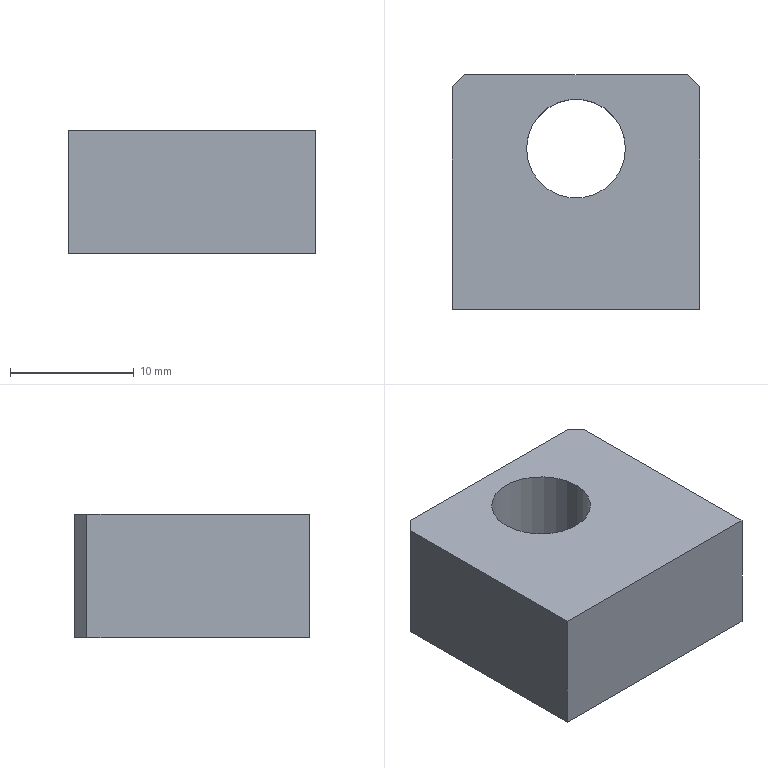Component | SolidWorks | LD101-02--Q1011-Q1-2-1 | 1 solid | 10 faces | box 20 x 19 x 10 mm | volume 3287 mm3 | plane 8 | cylinder 2 | commonest cylinder face diameters 8 x2 | material 45
build123d program:
from build123d import *

# Parameters (mm, degrees)
SKETCH1_W           = 20
SKETCH1_H           = 19
BOSS_EXTRUDE1_DEPTH = 5
SKETCH2_R           = 4
CUT_EXTRUDE1_DEPTH  = 12
CHAMFER1_SIZE       = 1


with BuildPart() as part:
    # Sketch1 → Boss-Extrude1 (new, symmetric)
    with BuildSketch(Plane.XY):
        Rectangle(SKETCH1_W, SKETCH1_H)
    extrude(amount=BOSS_EXTRUDE1_DEPTH, both=True)

    # Sketch2 → Cut-Extrude1 (cut)
    with BuildSketch(Plane.XY.offset(5)):
        with Locations((0, 3.5)):
            Circle(SKETCH2_R)
    extrude(amount=-CUT_EXTRUDE1_DEPTH, mode=Mode.SUBTRACT)

    # Chamfer1
    chamfer1_edges = [part.edges().sort_by_distance(p)[0] for p in [
        (-10, 9.5, 0),
        (10, 9.5, 0),
    ]]
    chamfer(chamfer1_edges, length=CHAMFER1_SIZE)


solid = part.part

# Placed as in the assembly
solid = solid.moved(Location((-360.29, -139.397, 162.257), (0, 0, 0)))
STEP:
#1=CARTESIAN_POINT('',(-14.027,-5.35,6.191));
#2=VERTEX_POINT('',#1);
#3=CARTESIAN_POINT('',(-14.342,-5.35,6.191));
#4=VERTEX_POINT('',#3);
#5=CARTESIAN_POINT('',(-14.185,-5.35,6.191));
#6=DIRECTION('',(0.,0.,-1.));
#7=DIRECTION('',(-1.,0.,0.));
#8=AXIS2_PLACEMENT_3D('',#5,#6,#7);
#9=CIRCLE('',#8,0.1575);
#10=EDGE_CURVE('',#2,#4,#9,.T.);
#11=ORIENTED_EDGE('',*,*,#10,.T.);
#12=CARTESIAN_POINT('',(-14.342,-5.35,6.585));
#13=VERTEX_POINT('',#12);
#14=CARTESIAN_POINT('',(-14.342,-5.35,6.112));
#15=DIRECTION('',(0.,0.,1.));
#16=VECTOR('',#15,39.37);
#17=LINE('',#14,#16);
#18=EDGE_CURVE('',#4,#13,#17,.T.);
#19=ORIENTED_EDGE('',*,*,#18,.T.);
#20=CARTESIAN_POINT('',(-14.027,-5.35,6.585));
#21=VERTEX_POINT('',#20);
#22=CARTESIAN_POINT('',(-14.185,-5.35,6.585));
#23=DIRECTION('',(0.,0.,1.));
#24=DIRECTION('',(1.,0.,0.));
#25=AXIS2_PLACEMENT_3D('',#22,#23,#24);
#26=CIRCLE('',#25,0.1575);
#27=EDGE_CURVE('',#13,#21,#26,.T.);
#28=ORIENTED_EDGE('',*,*,#27,.T.);
#29=CARTESIAN_POINT('',(-14.027,-5.35,6.112));
#30=DIRECTION('',(0.,0.,1.));
#31=VECTOR('',#30,39.37);
#32=LINE('',#29,#31);
#33=EDGE_CURVE('',#2,#21,#32,.T.);
#34=ORIENTED_EDGE('',*,*,#33,.F.);
#35=EDGE_LOOP('',(#11,#19,#28,#34));
#36=FACE_OUTER_BOUND('',#35,.T.);
#37=CARTESIAN_POINT('',(-14.185,-5.35,6.112));
#38=DIRECTION('',(0.,0.,1.));
#39=DIRECTION('',(1.,0.,0.));
#40=AXIS2_PLACEMENT_3D('',#37,#38,#39);
#41=CYLINDRICAL_SURFACE('',#40,0.1575);
#42=ADVANCED_FACE('',(#36),#41,.F.);
#43=CARTESIAN_POINT('',(-13.791,-5.862,6.191));
#44=VERTEX_POINT('',#43);
#45=CARTESIAN_POINT('',(-13.791,-5.153,6.191));
#46=VERTEX_POINT('',#45);
#47=CARTESIAN_POINT('',(-13.791,-5.862,6.191));
#48=DIRECTION('',(0.,1.,0.));
#49=VECTOR('',#48,39.37);
#50=LINE('',#47,#49);
#51=EDGE_CURVE('',#44,#46,#50,.T.);
#52=ORIENTED_EDGE('',*,*,#51,.T.);
#53=CARTESIAN_POINT('',(-13.791,-5.153,6.585));
#54=VERTEX_POINT('',#53);
#55=CARTESIAN_POINT('',(-13.791,-5.153,6.585));
#56=DIRECTION('',(0.,0.,1.));
#57=VECTOR('',#56,39.37);
#58=LINE('',#55,#57);
#59=EDGE_CURVE('',#46,#54,#58,.T.);
#60=ORIENTED_EDGE('',*,*,#59,.T.);
#61=CARTESIAN_POINT('',(-13.791,-5.862,6.585));
#62=VERTEX_POINT('',#61);
#63=CARTESIAN_POINT('',(-13.791,-5.862,6.585));
#64=DIRECTION('',(0.,1.,0.));
#65=VECTOR('',#64,39.37);
#66=LINE('',#63,#65);
#67=EDGE_CURVE('',#62,#54,#66,.T.);
#68=ORIENTED_EDGE('',*,*,#67,.F.);
#69=CARTESIAN_POINT('',(-13.791,-5.862,6.585));
#70=DIRECTION('',(0.,0.,-1.));
#71=VECTOR('',#70,39.37);
#72=LINE('',#69,#71);
#73=EDGE_CURVE('',#62,#44,#72,.T.);
#74=ORIENTED_EDGE('',*,*,#73,.T.);
#75=EDGE_LOOP('',(#52,#60,#68,#74));
#76=FACE_OUTER_BOUND('',#75,.T.);
#77=CARTESIAN_POINT('',(-13.791,-5.862,6.585));
#78=DIRECTION('',(-1.,0.,0.));
#79=DIRECTION('',(0.,0.,1.));
#80=AXIS2_PLACEMENT_3D('',#77,#78,#79);
#81=PLANE('',#80);
#82=ADVANCED_FACE('',(#76),#81,.F.);
#83=CARTESIAN_POINT('',(-13.83,-5.114,6.585));
#84=VERTEX_POINT('',#83);
#85=CARTESIAN_POINT('',(-14.539,-5.114,6.585));
#86=VERTEX_POINT('',#85);
#87=CARTESIAN_POINT('',(-14.578,-5.114,6.585));
#88=DIRECTION('',(-1.,0.,0.));
#89=VECTOR('',#88,39.37);
#90=LINE('',#87,#89);
#91=EDGE_CURVE('',#84,#86,#90,.T.);
#92=ORIENTED_EDGE('',*,*,#91,.F.);
#93=CARTESIAN_POINT('',(-13.83,-5.114,6.191));
#94=VERTEX_POINT('',#93);
#95=CARTESIAN_POINT('',(-13.83,-5.114,6.585));
#96=DIRECTION('',(0.,0.,-1.));
#97=VECTOR('',#96,39.37);
#98=LINE('',#95,#97);
#99=EDGE_CURVE('',#84,#94,#98,.T.);
#100=ORIENTED_EDGE('',*,*,#99,.T.);
#101=CARTESIAN_POINT('',(-14.539,-5.114,6.191));
#102=VERTEX_POINT('',#101);
#103=CARTESIAN_POINT('',(-14.578,-5.114,6.191));
#104=DIRECTION('',(-1.,0.,0.));
#105=VECTOR('',#104,39.37);
#106=LINE('',#103,#105);
#107=EDGE_CURVE('',#94,#102,#106,.T.);
#108=ORIENTED_EDGE('',*,*,#107,.T.);
#109=CARTESIAN_POINT('',(-14.539,-5.114,6.585));
#110=DIRECTION('',(0.,0.,1.));
#111=VECTOR('',#110,39.37);
#112=LINE('',#109,#111);
#113=EDGE_CURVE('',#102,#86,#112,.T.);
#114=ORIENTED_EDGE('',*,*,#113,.T.);
#115=EDGE_LOOP('',(#92,#100,#108,#114));
#116=FACE_OUTER_BOUND('',#115,.T.);
#117=CARTESIAN_POINT('',(-14.578,-5.114,6.585));
#118=DIRECTION('',(0.,-1.,0.));
#119=DIRECTION('',(0.,0.,-1.));
#120=AXIS2_PLACEMENT_3D('',#117,#118,#119);
#121=PLANE('',#120);
#122=ADVANCED_FACE('',(#116),#121,.F.);
#123=CARTESIAN_POINT('',(-14.578,-5.153,6.585));
#124=VERTEX_POINT('',#123);
#125=CARTESIAN_POINT('',(-14.578,-5.862,6.585));
#126=VERTEX_POINT('',#125);
#127=CARTESIAN_POINT('',(-14.578,-5.862,6.585));
#128=DIRECTION('',(0.,-1.,0.));
#129=VECTOR('',#128,39.37);
#130=LINE('',#127,#129);
#131=EDGE_CURVE('',#124,#126,#130,.T.);
#132=ORIENTED_EDGE('',*,*,#131,.F.);
#133=CARTESIAN_POINT('',(-14.578,-5.153,6.191));
#134=VERTEX_POINT('',#133);
#135=CARTESIAN_POINT('',(-14.578,-5.153,6.585));
#136=DIRECTION('',(0.,0.,-1.));
#137=VECTOR('',#136,39.37);
#138=LINE('',#135,#137);
#139=EDGE_CURVE('',#124,#134,#138,.T.);
#140=ORIENTED_EDGE('',*,*,#139,.T.);
#141=CARTESIAN_POINT('',(-14.578,-5.862,6.191));
#142=VERTEX_POINT('',#141);
#143=CARTESIAN_POINT('',(-14.578,-5.862,6.191));
#144=DIRECTION('',(0.,-1.,0.));
#145=VECTOR('',#144,39.37);
#146=LINE('',#143,#145);
#147=EDGE_CURVE('',#134,#142,#146,.T.);
#148=ORIENTED_EDGE('',*,*,#147,.T.);
#149=CARTESIAN_POINT('',(-14.578,-5.862,6.585));
#150=DIRECTION('',(0.,0.,-1.));
#151=VECTOR('',#150,39.37);
#152=LINE('',#149,#151);
#153=EDGE_CURVE('',#126,#142,#152,.T.);
#154=ORIENTED_EDGE('',*,*,#153,.F.);
#155=EDGE_LOOP('',(#132,#140,#148,#154));
#156=FACE_OUTER_BOUND('',#155,.T.);
#157=CARTESIAN_POINT('',(-14.578,-5.862,6.585));
#158=DIRECTION('',(1.,0.,0.));
#159=DIRECTION('',(0.,0.,-1.));
#160=AXIS2_PLACEMENT_3D('',#157,#158,#159);
#161=PLANE('',#160);
#162=ADVANCED_FACE('',(#156),#161,.F.);
#163=CARTESIAN_POINT('',(-14.578,-5.862,6.191));
#164=DIRECTION('',(1.,0.,0.));
#165=VECTOR('',#164,39.37);
#166=LINE('',#163,#165);
#167=EDGE_CURVE('',#142,#44,#166,.T.);
#168=ORIENTED_EDGE('',*,*,#167,.T.);
#169=ORIENTED_EDGE('',*,*,#73,.F.);
#170=CARTESIAN_POINT('',(-14.578,-5.862,6.585));
#171=DIRECTION('',(1.,0.,0.));
#172=VECTOR('',#171,39.37);
#173=LINE('',#170,#172);
#174=EDGE_CURVE('',#126,#62,#173,.T.);
#175=ORIENTED_EDGE('',*,*,#174,.F.);
#176=ORIENTED_EDGE('',*,*,#153,.T.);
#177=EDGE_LOOP('',(#168,#169,#175,#176));
#178=FACE_OUTER_BOUND('',#177,.T.);
#179=CARTESIAN_POINT('',(-14.578,-5.862,6.585));
#180=DIRECTION('',(0.,1.,0.));
#181=DIRECTION('',(0.,0.,1.));
#182=AXIS2_PLACEMENT_3D('',#179,#180,#181);
#183=PLANE('',#182);
#184=ADVANCED_FACE('',(#178),#183,.F.);
#185=CARTESIAN_POINT('',(-14.185,-5.35,6.585));
#186=DIRECTION('',(0.,0.,1.));
#187=DIRECTION('',(1.,0.,0.));
#188=AXIS2_PLACEMENT_3D('',#185,#186,#187);
#189=CIRCLE('',#188,0.1575);
#190=EDGE_CURVE('',#21,#13,#189,.T.);
#191=ORIENTED_EDGE('',*,*,#190,.F.);
#192=ORIENTED_EDGE('',*,*,#27,.F.);
#193=EDGE_LOOP('',(#191,#192));
#194=FACE_BOUND('',#193,.T.);
#195=ORIENTED_EDGE('',*,*,#67,.T.);
#196=CARTESIAN_POINT('',(-13.83,-5.114,6.585));
#197=DIRECTION('',(-0.7071,0.7071,0.));
#198=VECTOR('',#197,39.37);
#199=LINE('',#196,#198);
#200=EDGE_CURVE('',#54,#84,#199,.T.);
#201=ORIENTED_EDGE('',*,*,#200,.T.);
#202=ORIENTED_EDGE('',*,*,#91,.T.);
#203=CARTESIAN_POINT('',(-14.578,-5.153,6.585));
#204=DIRECTION('',(-0.7071,-0.7071,0.));
#205=VECTOR('',#204,39.37);
#206=LINE('',#203,#205);
#207=EDGE_CURVE('',#86,#124,#206,.T.);
#208=ORIENTED_EDGE('',*,*,#207,.T.);
#209=ORIENTED_EDGE('',*,*,#131,.T.);
#210=ORIENTED_EDGE('',*,*,#174,.T.);
#211=EDGE_LOOP('',(#195,#201,#202,#208,#209,#210));
#212=FACE_OUTER_BOUND('',#211,.T.);
#213=CARTESIAN_POINT('',(-14.185,-5.488,6.585));
#214=DIRECTION('',(0.,0.,-1.));
#215=DIRECTION('',(-1.,0.,0.));
#216=AXIS2_PLACEMENT_3D('',#213,#214,#215);
#217=PLANE('',#216);
#218=ADVANCED_FACE('',(#194,#212),#217,.F.);
#219=ORIENTED_EDGE('',*,*,#10,.F.);
#220=CARTESIAN_POINT('',(-14.185,-5.35,6.191));
#221=DIRECTION('',(0.,0.,-1.));
#222=DIRECTION('',(-1.,0.,0.));
#223=AXIS2_PLACEMENT_3D('',#220,#221,#222);
#224=CIRCLE('',#223,0.1575);
#225=EDGE_CURVE('',#4,#2,#224,.T.);
#226=ORIENTED_EDGE('',*,*,#225,.F.);
#227=EDGE_LOOP('',(#219,#226));
#228=FACE_BOUND('',#227,.T.);
#229=ORIENTED_EDGE('',*,*,#107,.F.);
#230=CARTESIAN_POINT('',(-13.82,-5.124,6.191));
#231=DIRECTION('',(0.7071,-0.7071,0.));
#232=VECTOR('',#231,39.37);
#233=LINE('',#230,#232);
#234=EDGE_CURVE('',#94,#46,#233,.T.);
#235=ORIENTED_EDGE('',*,*,#234,.T.);
#236=ORIENTED_EDGE('',*,*,#51,.F.);
#237=ORIENTED_EDGE('',*,*,#167,.F.);
#238=ORIENTED_EDGE('',*,*,#147,.F.);
#239=CARTESIAN_POINT('',(-14.549,-5.124,6.191));
#240=DIRECTION('',(0.7071,0.7071,0.));
#241=VECTOR('',#240,39.37);
#242=LINE('',#239,#241);
#243=EDGE_CURVE('',#134,#102,#242,.T.);
#244=ORIENTED_EDGE('',*,*,#243,.T.);
#245=EDGE_LOOP('',(#229,#235,#236,#237,#238,#244));
#246=FACE_OUTER_BOUND('',#245,.T.);
#247=CARTESIAN_POINT('',(-14.185,-5.488,6.191));
#248=DIRECTION('',(0.,0.,-1.));
#249=DIRECTION('',(-1.,0.,0.));
#250=AXIS2_PLACEMENT_3D('',#247,#248,#249);
#251=PLANE('',#250);
#252=ADVANCED_FACE('',(#228,#246),#251,.T.);
#253=ORIENTED_EDGE('',*,*,#18,.F.);
#254=ORIENTED_EDGE('',*,*,#225,.T.);
#255=ORIENTED_EDGE('',*,*,#33,.T.);
#256=ORIENTED_EDGE('',*,*,#190,.T.);
#257=EDGE_LOOP('',(#253,#254,#255,#256));
#258=FACE_OUTER_BOUND('',#257,.T.);
#259=CARTESIAN_POINT('',(-14.185,-5.35,6.112));
#260=DIRECTION('',(0.,0.,1.));
#261=DIRECTION('',(1.,0.,0.));
#262=AXIS2_PLACEMENT_3D('',#259,#260,#261);
#263=CYLINDRICAL_SURFACE('',#262,0.1575);
#264=ADVANCED_FACE('',(#258),#263,.F.);
#265=ORIENTED_EDGE('',*,*,#200,.F.);
#266=ORIENTED_EDGE('',*,*,#59,.F.);
#267=ORIENTED_EDGE('',*,*,#234,.F.);
#268=ORIENTED_EDGE('',*,*,#99,.F.);
#269=EDGE_LOOP('',(#265,#266,#267,#268));
#270=FACE_OUTER_BOUND('',#269,.T.);
#271=CARTESIAN_POINT('',(-13.83,-5.114,6.585));
#272=DIRECTION('',(-0.7071,-0.7071,0.));
#273=DIRECTION('',(0.,0.,-1.));
#274=AXIS2_PLACEMENT_3D('',#271,#272,#273);
#275=PLANE('',#274);
#276=ADVANCED_FACE('',(#270),#275,.F.);
#277=ORIENTED_EDGE('',*,*,#207,.F.);
#278=ORIENTED_EDGE('',*,*,#113,.F.);
#279=ORIENTED_EDGE('',*,*,#243,.F.);
#280=ORIENTED_EDGE('',*,*,#139,.F.);
#281=EDGE_LOOP('',(#277,#278,#279,#280));
#282=FACE_OUTER_BOUND('',#281,.T.);
#283=CARTESIAN_POINT('',(-14.578,-5.153,6.585));
#284=DIRECTION('',(0.7071,-0.7071,0.));
#285=DIRECTION('',(0.,0.,-1.));
#286=AXIS2_PLACEMENT_3D('',#283,#284,#285);
#287=PLANE('',#286);
#288=ADVANCED_FACE('',(#282),#287,.F.);
#289=CLOSED_SHELL('',(#42,#82,#122,#162,#184,#218,#252,#264,#276,#288));
#290=MANIFOLD_SOLID_BREP('',#289);
#291=CARTESIAN_POINT('',(0.,0.,0.));
#292=DIRECTION('',(0.,0.,1.));
#293=DIRECTION('',(1.,0.,0.));
#294=AXIS2_PLACEMENT_3D('',#291,#292,#293);
#295=(LENGTH_UNIT()NAMED_UNIT(*)SI_UNIT($,.METRE.));
#296=LENGTH_MEASURE_WITH_UNIT(LENGTH_MEASURE(0.0254),#295);
#297=DIMENSIONAL_EXPONENTS(1.,0.,0.,0.,0.,0.,0.);
#298=(CONVERSION_BASED_UNIT('',#296)LENGTH_UNIT()NAMED_UNIT(#297));
#299=UNCERTAINTY_MEASURE_WITH_UNIT(LENGTH_MEASURE(0.00001),#298,'','');
#300=(NAMED_UNIT(*)PLANE_ANGLE_UNIT()SI_UNIT($,.RADIAN.));
#301=(NAMED_UNIT(*)SI_UNIT($,.STERADIAN.)SOLID_ANGLE_UNIT());
#302=(GEOMETRIC_REPRESENTATION_CONTEXT(3)GLOBAL_UNCERTAINTY_ASSIGNED_CONTEXT((#299))GLOBAL_UNIT_ASSIGNED_CONTEXT((#298,#300,#301))REPRESENTATION_CONTEXT('',''));
#303=ADVANCED_BREP_SHAPE_REPRESENTATION('',(#290,#294),#302);
#304=COLOUR_RGB('',0.7922,0.8196,0.9333);
#305=FILL_AREA_STYLE_COLOUR('',#304);
#306=FILL_AREA_STYLE('',(#305));
#307=SURFACE_STYLE_FILL_AREA(#306);
#308=SURFACE_SIDE_STYLE('',(#307));
#309=SURFACE_STYLE_USAGE(.BOTH.,#308);
#310=PRESENTATION_STYLE_ASSIGNMENT((#309));
#311=STYLED_ITEM('',(#310),#290);
#312=(LENGTH_UNIT()NAMED_UNIT(*)SI_UNIT($,.METRE.));
#313=LENGTH_MEASURE_WITH_UNIT(LENGTH_MEASURE(0.0254),#312);
#314=DIMENSIONAL_EXPONENTS(1.,0.,0.,0.,0.,0.,0.);
#315=(CONVERSION_BASED_UNIT('',#313)LENGTH_UNIT()NAMED_UNIT(#314));
#316=UNCERTAINTY_MEASURE_WITH_UNIT(LENGTH_MEASURE(0.00001),#315,'','');
#317=(NAMED_UNIT(*)PLANE_ANGLE_UNIT()SI_UNIT($,.RADIAN.));
#318=(NAMED_UNIT(*)SI_UNIT($,.STERADIAN.)SOLID_ANGLE_UNIT());
#319=(GEOMETRIC_REPRESENTATION_CONTEXT(3)GLOBAL_UNCERTAINTY_ASSIGNED_CONTEXT((#316))GLOBAL_UNIT_ASSIGNED_CONTEXT((#315,#317,#318))REPRESENTATION_CONTEXT('',''));
#320=MECHANICAL_DESIGN_GEOMETRIC_PRESENTATION_REPRESENTATION('',(#311),#319);
#321=PRESENTATION_LAYER_ASSIGNMENT('','',(#311));